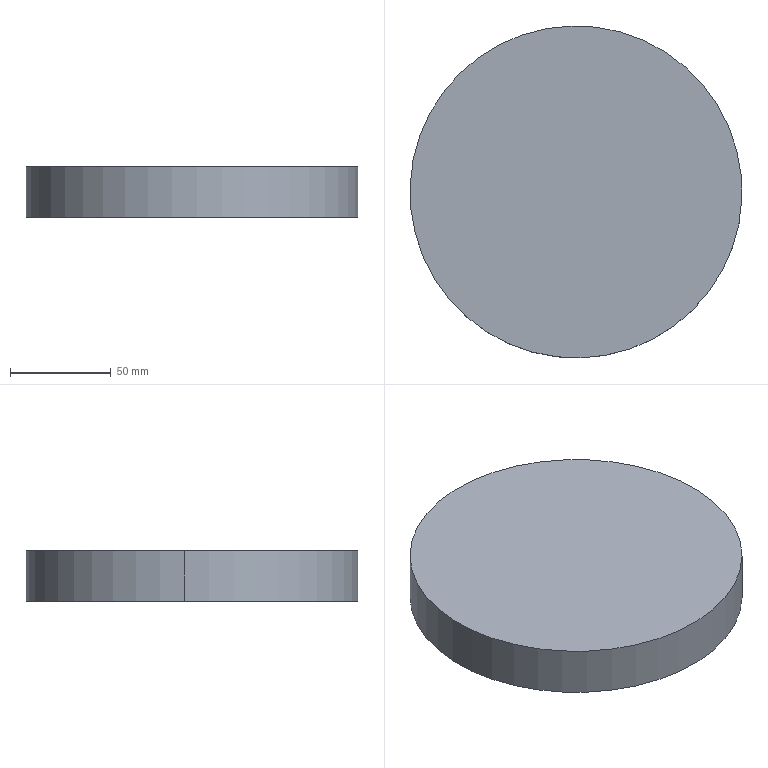Component | SolidWorks | PunchPad-1 | 1 solid | 4 faces | box 165 x 165 x 25 mm | volume 534562 mm3 | cylinder 2 | plane 2 | commonest cylinder face diameters 165 x2
build123d program:
from build123d import *

# Parameters (mm, degrees)
SKETCH1_R           = 82.5
BOSS_EXTRUDE1_DEPTH = 25


with BuildPart() as part:
    # Sketch1 → Boss-Extrude1 (new body)
    with BuildSketch(Plane.XY):
        Circle(SKETCH1_R)
    extrude(amount=BOSS_EXTRUDE1_DEPTH)


solid = part.part

# Placed as in the assembly
solid = solid.moved(Location((0, 0, -271), (0, 0, 0)))
STEP:
#1=CARTESIAN_POINT('',(3.245,-0.145,-9.685));
#2=VERTEX_POINT('',#1);
#3=CARTESIAN_POINT('',(-3.245,0.145,-9.685));
#4=VERTEX_POINT('',#3);
#5=CARTESIAN_POINT('',(-0.,0.,-9.685));
#6=DIRECTION('',(0.,0.,1.));
#7=DIRECTION('',(0.999,-0.04464,0.));
#8=AXIS2_PLACEMENT_3D('',#5,#6,#7);
#9=CIRCLE('',#8,3.248);
#10=EDGE_CURVE('',#2,#4,#9,.T.);
#11=ORIENTED_EDGE('',*,*,#10,.F.);
#12=CARTESIAN_POINT('',(3.245,-0.145,-10.669));
#13=VERTEX_POINT('',#12);
#14=CARTESIAN_POINT('',(3.245,-0.145,-9.685));
#15=DIRECTION('',(0.,0.,-1.));
#16=VECTOR('',#15,39.37);
#17=LINE('',#14,#16);
#18=EDGE_CURVE('',#2,#13,#17,.T.);
#19=ORIENTED_EDGE('',*,*,#18,.T.);
#20=CARTESIAN_POINT('',(-3.245,0.145,-10.669));
#21=VERTEX_POINT('',#20);
#22=CARTESIAN_POINT('',(-0.,0.,-10.669));
#23=DIRECTION('',(0.,0.,1.));
#24=DIRECTION('',(0.999,-0.04464,0.));
#25=AXIS2_PLACEMENT_3D('',#22,#23,#24);
#26=CIRCLE('',#25,3.248);
#27=EDGE_CURVE('',#13,#21,#26,.T.);
#28=ORIENTED_EDGE('',*,*,#27,.T.);
#29=CARTESIAN_POINT('',(-3.245,0.145,-9.685));
#30=DIRECTION('',(0.,0.,-1.));
#31=VECTOR('',#30,39.37);
#32=LINE('',#29,#31);
#33=EDGE_CURVE('',#4,#21,#32,.T.);
#34=ORIENTED_EDGE('',*,*,#33,.F.);
#35=EDGE_LOOP('',(#11,#19,#28,#34));
#36=FACE_OUTER_BOUND('',#35,.T.);
#37=CARTESIAN_POINT('',(-0.,0.,-9.685));
#38=DIRECTION('',(0.,0.,-1.));
#39=DIRECTION('',(-0.999,0.04464,0.));
#40=AXIS2_PLACEMENT_3D('',#37,#38,#39);
#41=CYLINDRICAL_SURFACE('',#40,3.248);
#42=ADVANCED_FACE('',(#36),#41,.T.);
#43=ORIENTED_EDGE('',*,*,#18,.F.);
#44=CARTESIAN_POINT('',(-0.,0.,-9.685));
#45=DIRECTION('',(0.,0.,1.));
#46=DIRECTION('',(0.999,-0.04464,0.));
#47=AXIS2_PLACEMENT_3D('',#44,#45,#46);
#48=CIRCLE('',#47,3.248);
#49=EDGE_CURVE('',#4,#2,#48,.T.);
#50=ORIENTED_EDGE('',*,*,#49,.F.);
#51=ORIENTED_EDGE('',*,*,#33,.T.);
#52=CARTESIAN_POINT('',(-0.,0.,-10.669));
#53=DIRECTION('',(0.,0.,1.));
#54=DIRECTION('',(0.999,-0.04464,0.));
#55=AXIS2_PLACEMENT_3D('',#52,#53,#54);
#56=CIRCLE('',#55,3.248);
#57=EDGE_CURVE('',#21,#13,#56,.T.);
#58=ORIENTED_EDGE('',*,*,#57,.T.);
#59=EDGE_LOOP('',(#43,#50,#51,#58));
#60=FACE_OUTER_BOUND('',#59,.T.);
#61=CARTESIAN_POINT('',(-0.,0.,-9.685));
#62=DIRECTION('',(0.,0.,-1.));
#63=DIRECTION('',(-0.999,0.04464,0.));
#64=AXIS2_PLACEMENT_3D('',#61,#62,#63);
#65=CYLINDRICAL_SURFACE('',#64,3.248);
#66=ADVANCED_FACE('',(#60),#65,.T.);
#67=ORIENTED_EDGE('',*,*,#49,.T.);
#68=ORIENTED_EDGE('',*,*,#10,.T.);
#69=EDGE_LOOP('',(#67,#68));
#70=FACE_OUTER_BOUND('',#69,.T.);
#71=CARTESIAN_POINT('',(-0.,0.,-9.685));
#72=DIRECTION('',(0.,0.,1.));
#73=DIRECTION('',(0.999,-0.04464,0.));
#74=AXIS2_PLACEMENT_3D('',#71,#72,#73);
#75=PLANE('',#74);
#76=ADVANCED_FACE('',(#70),#75,.T.);
#77=ORIENTED_EDGE('',*,*,#57,.F.);
#78=ORIENTED_EDGE('',*,*,#27,.F.);
#79=EDGE_LOOP('',(#77,#78));
#80=FACE_OUTER_BOUND('',#79,.T.);
#81=CARTESIAN_POINT('',(-0.,0.,-10.669));
#82=DIRECTION('',(0.,0.,1.));
#83=DIRECTION('',(0.999,-0.04464,0.));
#84=AXIS2_PLACEMENT_3D('',#81,#82,#83);
#85=PLANE('',#84);
#86=ADVANCED_FACE('',(#80),#85,.F.);
#87=CLOSED_SHELL('',(#42,#66,#76,#86));
#88=MANIFOLD_SOLID_BREP('',#87);
#89=CARTESIAN_POINT('',(0.,0.,0.));
#90=DIRECTION('',(0.,0.,1.));
#91=DIRECTION('',(1.,0.,0.));
#92=AXIS2_PLACEMENT_3D('',#89,#90,#91);
#93=(LENGTH_UNIT()NAMED_UNIT(*)SI_UNIT($,.METRE.));
#94=LENGTH_MEASURE_WITH_UNIT(LENGTH_MEASURE(0.0254),#93);
#95=DIMENSIONAL_EXPONENTS(1.,0.,0.,0.,0.,0.,0.);
#96=(CONVERSION_BASED_UNIT('',#94)LENGTH_UNIT()NAMED_UNIT(#95));
#97=UNCERTAINTY_MEASURE_WITH_UNIT(LENGTH_MEASURE(0.00001),#96,'','');
#98=(NAMED_UNIT(*)PLANE_ANGLE_UNIT()SI_UNIT($,.RADIAN.));
#99=(NAMED_UNIT(*)SI_UNIT($,.STERADIAN.)SOLID_ANGLE_UNIT());
#100=(GEOMETRIC_REPRESENTATION_CONTEXT(3)GLOBAL_UNCERTAINTY_ASSIGNED_CONTEXT((#97))GLOBAL_UNIT_ASSIGNED_CONTEXT((#96,#98,#99))REPRESENTATION_CONTEXT('',''));
#101=ADVANCED_BREP_SHAPE_REPRESENTATION('',(#88,#92),#100);
#102=COLOUR_RGB('',0.7922,0.8196,0.9333);
#103=FILL_AREA_STYLE_COLOUR('',#102);
#104=FILL_AREA_STYLE('',(#103));
#105=SURFACE_STYLE_FILL_AREA(#104);
#106=SURFACE_SIDE_STYLE('',(#105));
#107=SURFACE_STYLE_USAGE(.BOTH.,#106);
#108=PRESENTATION_STYLE_ASSIGNMENT((#107));
#109=STYLED_ITEM('',(#108),#88);
#110=PRESENTATION_LAYER_ASSIGNMENT('','',(#109));
#111=(LENGTH_UNIT()NAMED_UNIT(*)SI_UNIT($,.METRE.));
#112=LENGTH_MEASURE_WITH_UNIT(LENGTH_MEASURE(0.0254),#111);
#113=DIMENSIONAL_EXPONENTS(1.,0.,0.,0.,0.,0.,0.);
#114=(CONVERSION_BASED_UNIT('',#112)LENGTH_UNIT()NAMED_UNIT(#113));
#115=UNCERTAINTY_MEASURE_WITH_UNIT(LENGTH_MEASURE(0.00001),#114,'','');
#116=(NAMED_UNIT(*)PLANE_ANGLE_UNIT()SI_UNIT($,.RADIAN.));
#117=(NAMED_UNIT(*)SI_UNIT($,.STERADIAN.)SOLID_ANGLE_UNIT());
#118=(GEOMETRIC_REPRESENTATION_CONTEXT(3)GLOBAL_UNCERTAINTY_ASSIGNED_CONTEXT((#115))GLOBAL_UNIT_ASSIGNED_CONTEXT((#114,#116,#117))REPRESENTATION_CONTEXT('',''));
#119=MECHANICAL_DESIGN_GEOMETRIC_PRESENTATION_REPRESENTATION('',(#109),#118);